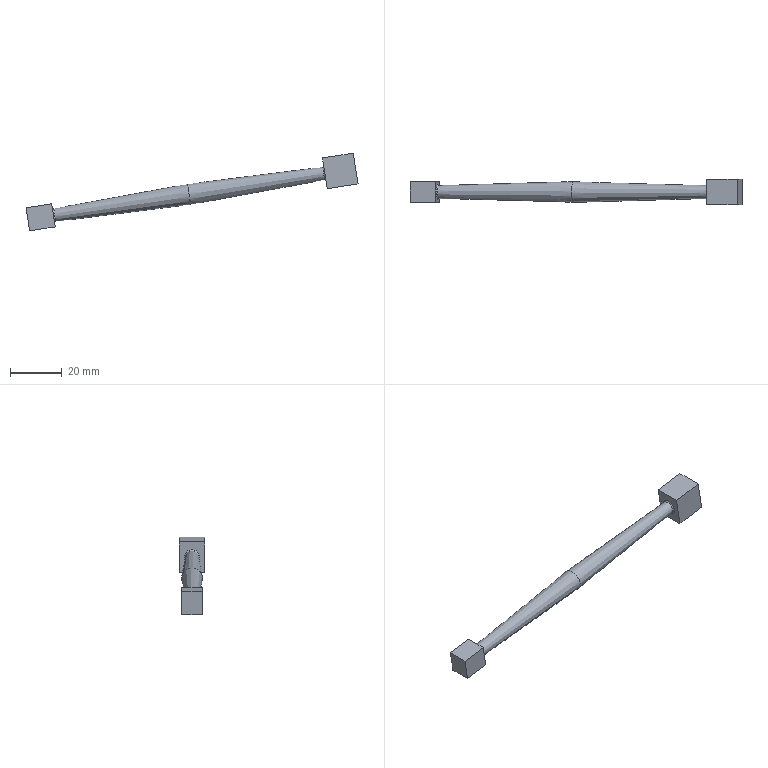Component | NX | LINK_1 | 1 solid | 17 faces | volume 5742 mm3 | plane 12 | torus 3 | cone 2